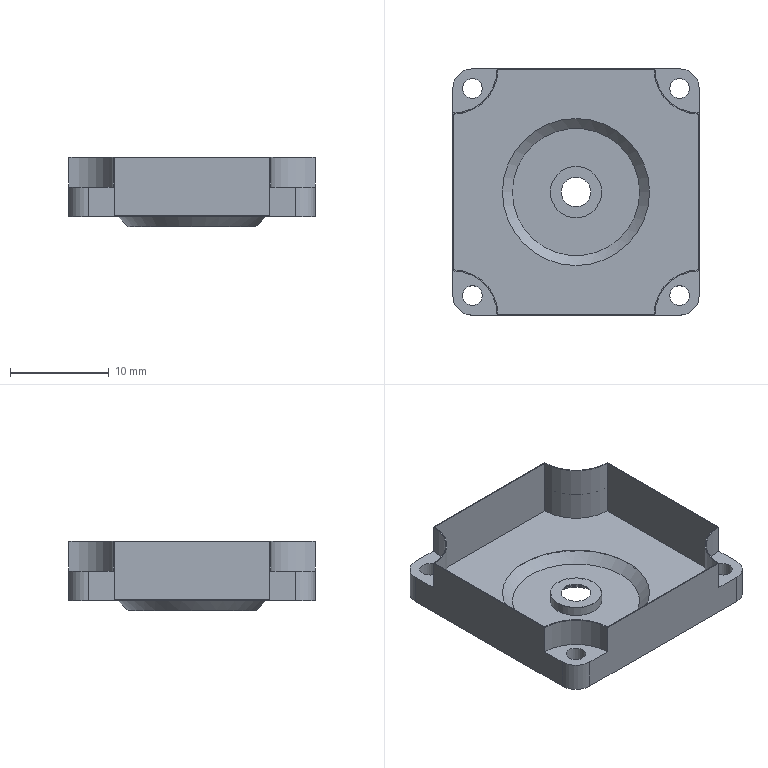Component | NX | STEPPER_FRONT | 1 solid | 40 faces | volume 256 mm3 | cylinder 19 | plane 19 | cone 2 | commonest cylinder face diameters 9 x4 2 x4 4 x4 9.2 x4 3 x1 5 x1 5.2 x1